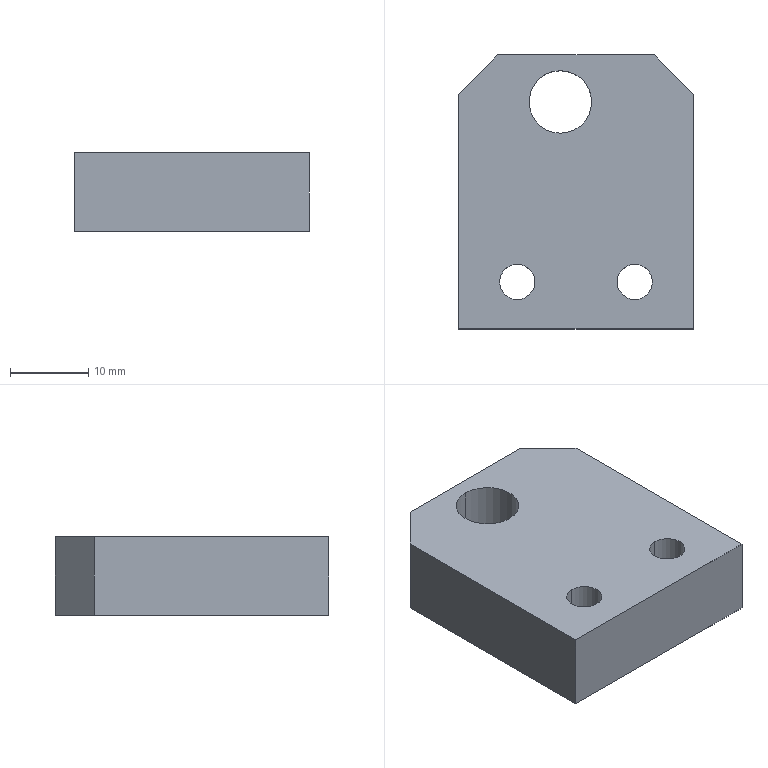Component | SolidWorks | LSDH-6-029-1 | 1 solid | 20 faces | box 30 x 35 x 10 mm | volume 9113 mm3 | cylinder 10 | plane 10 | commonest cylinder face diameters 8 x6 4.5 x4
build123d program:
from build123d import *

# Parameters (mm, degrees)
SKETCH1_W                                            = 35
SKETCH1_H                                            = 30
BOSS_EXTRUDE1_DEPTH                                  = 10
M8X1_0_TAPPED_HOLE1_D                                = 8
M8X1_0_TAPPED_HOLE1_DEPTH                            = 19
M8X1_0_TAPPED_HOLE1_TIP                              = 2.403
HOLE_SIZE_ACCORDING_TO_THE_TYPE_OF_HEX_S_D           = 4.5
HOLE_SIZE_ACCORDING_TO_THE_TYPE_OF_HEX_S_CBORE_D     = 8
HOLE_SIZE_ACCORDING_TO_THE_TYPE_OF_HEX_S_CBORE_DEPTH = 4.6
CHAMFER1_SIZE                                        = 5


with BuildPart() as part:
    # Sketch1 → Boss-Extrude1 (new body)
    with BuildSketch(Plane.XY):
        Rectangle(SKETCH1_W, SKETCH1_H)
    extrude(amount=BOSS_EXTRUDE1_DEPTH)

    # M8x1.0 Tapped Hole1
    with Locations(Plane(origin=(11.5, 2, 10), x_dir=(1, 0, 0), z_dir=(0, 0, 1))):
        with Locations((0, 0)):
            Hole(M8X1_0_TAPPED_HOLE1_D / 2, depth=M8X1_0_TAPPED_HOLE1_DEPTH)
            with Locations((0, 0, -(M8X1_0_TAPPED_HOLE1_DEPTH + M8X1_0_TAPPED_HOLE1_TIP / 2))):  # 118° drill point
                Cone(0, M8X1_0_TAPPED_HOLE1_D / 2, M8X1_0_TAPPED_HOLE1_TIP, mode=Mode.SUBTRACT)

    # Hole size according to the type of hex s (through all)
    with Locations(Plane(origin=(-11.5, 7.5, 0), x_dir=(-1, 0, 0), z_dir=(0, 0, -1))):
        with Locations((0, 0), (0, -15)):
            CounterBoreHole(HOLE_SIZE_ACCORDING_TO_THE_TYPE_OF_HEX_S_D / 2, HOLE_SIZE_ACCORDING_TO_THE_TYPE_OF_HEX_S_CBORE_D / 2, HOLE_SIZE_ACCORDING_TO_THE_TYPE_OF_HEX_S_CBORE_DEPTH)

    # Chamfer1
    chamfer1_edges = [part.edges().sort_by_distance(p)[0] for p in [
        (17.5, -15, 5),
        (17.5, 15, 5),
    ]]
    chamfer(chamfer1_edges, length=CHAMFER1_SIZE)


solid = part.part

# Placed as in the assembly
solid = solid.moved(Location((274.305, 297.675, 54.479), (0, 0, 90)))
STEP:
#1=COLOUR_RGB('',0.7922,0.8196,0.9333);
#2=FILL_AREA_STYLE_COLOUR('',#1);
#3=FILL_AREA_STYLE('',(#2));
#4=SURFACE_STYLE_FILL_AREA(#3);
#5=SURFACE_SIDE_STYLE('',(#4));
#6=SURFACE_STYLE_USAGE(.BOTH.,#5);
#7=PRESENTATION_STYLE_ASSIGNMENT((#6));
#8=CARTESIAN_POINT('',(10.504,11.424,2.326));
#9=VERTEX_POINT('',#8);
#10=CARTESIAN_POINT('',(10.504,11.109,2.326));
#11=VERTEX_POINT('',#10);
#12=CARTESIAN_POINT('',(10.504,11.267,2.326));
#13=DIRECTION('',(0.,-0.,-1.));
#14=DIRECTION('',(0.,-1.,0.));
#15=AXIS2_PLACEMENT_3D('',#12,#13,#14);
#16=CIRCLE('',#15,0.1575);
#17=EDGE_CURVE('',#9,#11,#16,.T.);
#18=ORIENTED_EDGE('',*,*,#17,.F.);
#19=CARTESIAN_POINT('',(10.504,11.424,2.145));
#20=VERTEX_POINT('',#19);
#21=CARTESIAN_POINT('',(10.504,11.424,2.145));
#22=DIRECTION('',(0.,-0.,-1.));
#23=VECTOR('',#22,39.37);
#24=LINE('',#21,#23);
#25=EDGE_CURVE('',#9,#20,#24,.T.);
#26=ORIENTED_EDGE('',*,*,#25,.T.);
#27=CARTESIAN_POINT('',(10.504,11.109,2.145));
#28=VERTEX_POINT('',#27);
#29=CARTESIAN_POINT('',(10.504,11.267,2.145));
#30=DIRECTION('',(0.,-0.,-1.));
#31=DIRECTION('',(0.,-1.,0.));
#32=AXIS2_PLACEMENT_3D('',#29,#30,#31);
#33=CIRCLE('',#32,0.1575);
#34=EDGE_CURVE('',#20,#28,#33,.T.);
#35=ORIENTED_EDGE('',*,*,#34,.T.);
#36=CARTESIAN_POINT('',(10.504,11.109,2.145));
#37=DIRECTION('',(0.,-0.,-1.));
#38=VECTOR('',#37,39.37);
#39=LINE('',#36,#38);
#40=EDGE_CURVE('',#11,#28,#39,.T.);
#41=ORIENTED_EDGE('',*,*,#40,.F.);
#42=EDGE_LOOP('',(#18,#26,#35,#41));
#43=FACE_OUTER_BOUND('',#42,.T.);
#44=CARTESIAN_POINT('',(10.504,11.267,2.145));
#45=DIRECTION('',(0.,-0.,-1.));
#46=DIRECTION('',(0.,-1.,0.));
#47=AXIS2_PLACEMENT_3D('',#44,#45,#46);
#48=CYLINDRICAL_SURFACE('',#47,0.1575);
#49=ADVANCED_FACE('',(#43),#48,.F.);
#50=CARTESIAN_POINT('',(10.504,11.355,2.539));
#51=VERTEX_POINT('',#50);
#52=CARTESIAN_POINT('',(10.504,11.178,2.539));
#53=VERTEX_POINT('',#52);
#54=CARTESIAN_POINT('',(10.504,11.267,2.539));
#55=DIRECTION('',(0.,-0.,-1.));
#56=DIRECTION('',(0.,-1.,0.));
#57=AXIS2_PLACEMENT_3D('',#54,#55,#56);
#58=CIRCLE('',#57,0.08858);
#59=EDGE_CURVE('',#51,#53,#58,.T.);
#60=ORIENTED_EDGE('',*,*,#59,.F.);
#61=CARTESIAN_POINT('',(10.504,11.355,2.326));
#62=VERTEX_POINT('',#61);
#63=CARTESIAN_POINT('',(10.504,11.355,2.145));
#64=DIRECTION('',(0.,-0.,-1.));
#65=VECTOR('',#64,39.37);
#66=LINE('',#63,#65);
#67=EDGE_CURVE('',#51,#62,#66,.T.);
#68=ORIENTED_EDGE('',*,*,#67,.T.);
#69=CARTESIAN_POINT('',(10.504,11.178,2.326));
#70=VERTEX_POINT('',#69);
#71=CARTESIAN_POINT('',(10.504,11.267,2.326));
#72=DIRECTION('',(0.,-0.,-1.));
#73=DIRECTION('',(0.,-1.,0.));
#74=AXIS2_PLACEMENT_3D('',#71,#72,#73);
#75=CIRCLE('',#74,0.08858);
#76=EDGE_CURVE('',#62,#70,#75,.T.);
#77=ORIENTED_EDGE('',*,*,#76,.T.);
#78=CARTESIAN_POINT('',(10.504,11.178,2.145));
#79=DIRECTION('',(0.,-0.,-1.));
#80=VECTOR('',#79,39.37);
#81=LINE('',#78,#80);
#82=EDGE_CURVE('',#53,#70,#81,.T.);
#83=ORIENTED_EDGE('',*,*,#82,.F.);
#84=EDGE_LOOP('',(#60,#68,#77,#83));
#85=FACE_OUTER_BOUND('',#84,.T.);
#86=CARTESIAN_POINT('',(10.504,11.267,2.145));
#87=DIRECTION('',(0.,-0.,-1.));
#88=DIRECTION('',(0.,-1.,0.));
#89=AXIS2_PLACEMENT_3D('',#86,#87,#88);
#90=CYLINDRICAL_SURFACE('',#89,0.08858);
#91=ADVANCED_FACE('',(#85),#90,.F.);
#92=CARTESIAN_POINT('',(11.095,11.424,2.326));
#93=VERTEX_POINT('',#92);
#94=CARTESIAN_POINT('',(11.095,11.109,2.326));
#95=VERTEX_POINT('',#94);
#96=CARTESIAN_POINT('',(11.095,11.267,2.326));
#97=DIRECTION('',(0.,-0.,-1.));
#98=DIRECTION('',(0.,-1.,0.));
#99=AXIS2_PLACEMENT_3D('',#96,#97,#98);
#100=CIRCLE('',#99,0.1575);
#101=EDGE_CURVE('',#93,#95,#100,.T.);
#102=ORIENTED_EDGE('',*,*,#101,.F.);
#103=CARTESIAN_POINT('',(11.095,11.424,2.145));
#104=VERTEX_POINT('',#103);
#105=CARTESIAN_POINT('',(11.095,11.424,2.145));
#106=DIRECTION('',(0.,-0.,-1.));
#107=VECTOR('',#106,39.37);
#108=LINE('',#105,#107);
#109=EDGE_CURVE('',#93,#104,#108,.T.);
#110=ORIENTED_EDGE('',*,*,#109,.T.);
#111=CARTESIAN_POINT('',(11.095,11.109,2.145));
#112=VERTEX_POINT('',#111);
#113=CARTESIAN_POINT('',(11.095,11.267,2.145));
#114=DIRECTION('',(0.,-0.,-1.));
#115=DIRECTION('',(0.,-1.,0.));
#116=AXIS2_PLACEMENT_3D('',#113,#114,#115);
#117=CIRCLE('',#116,0.1575);
#118=EDGE_CURVE('',#104,#112,#117,.T.);
#119=ORIENTED_EDGE('',*,*,#118,.T.);
#120=CARTESIAN_POINT('',(11.095,11.109,2.145));
#121=DIRECTION('',(0.,-0.,-1.));
#122=VECTOR('',#121,39.37);
#123=LINE('',#120,#122);
#124=EDGE_CURVE('',#95,#112,#123,.T.);
#125=ORIENTED_EDGE('',*,*,#124,.F.);
#126=EDGE_LOOP('',(#102,#110,#119,#125));
#127=FACE_OUTER_BOUND('',#126,.T.);
#128=CARTESIAN_POINT('',(11.095,11.267,2.145));
#129=DIRECTION('',(0.,-0.,-1.));
#130=DIRECTION('',(0.,-1.,0.));
#131=AXIS2_PLACEMENT_3D('',#128,#129,#130);
#132=CYLINDRICAL_SURFACE('',#131,0.1575);
#133=ADVANCED_FACE('',(#127),#132,.F.);
#134=CARTESIAN_POINT('',(11.095,11.355,2.539));
#135=VERTEX_POINT('',#134);
#136=CARTESIAN_POINT('',(11.095,11.178,2.539));
#137=VERTEX_POINT('',#136);
#138=CARTESIAN_POINT('',(11.095,11.267,2.539));
#139=DIRECTION('',(0.,-0.,-1.));
#140=DIRECTION('',(0.,-1.,0.));
#141=AXIS2_PLACEMENT_3D('',#138,#139,#140);
#142=CIRCLE('',#141,0.08858);
#143=EDGE_CURVE('',#135,#137,#142,.T.);
#144=ORIENTED_EDGE('',*,*,#143,.F.);
#145=CARTESIAN_POINT('',(11.095,11.355,2.326));
#146=VERTEX_POINT('',#145);
#147=CARTESIAN_POINT('',(11.095,11.355,2.145));
#148=DIRECTION('',(0.,-0.,-1.));
#149=VECTOR('',#148,39.37);
#150=LINE('',#147,#149);
#151=EDGE_CURVE('',#135,#146,#150,.T.);
#152=ORIENTED_EDGE('',*,*,#151,.T.);
#153=CARTESIAN_POINT('',(11.095,11.178,2.326));
#154=VERTEX_POINT('',#153);
#155=CARTESIAN_POINT('',(11.095,11.267,2.326));
#156=DIRECTION('',(0.,-0.,-1.));
#157=DIRECTION('',(0.,-1.,0.));
#158=AXIS2_PLACEMENT_3D('',#155,#156,#157);
#159=CIRCLE('',#158,0.08858);
#160=EDGE_CURVE('',#146,#154,#159,.T.);
#161=ORIENTED_EDGE('',*,*,#160,.T.);
#162=CARTESIAN_POINT('',(11.095,11.178,2.145));
#163=DIRECTION('',(0.,-0.,-1.));
#164=VECTOR('',#163,39.37);
#165=LINE('',#162,#164);
#166=EDGE_CURVE('',#137,#154,#165,.T.);
#167=ORIENTED_EDGE('',*,*,#166,.F.);
#168=EDGE_LOOP('',(#144,#152,#161,#167));
#169=FACE_OUTER_BOUND('',#168,.T.);
#170=CARTESIAN_POINT('',(11.095,11.267,2.145));
#171=DIRECTION('',(0.,-0.,-1.));
#172=DIRECTION('',(0.,-1.,0.));
#173=AXIS2_PLACEMENT_3D('',#170,#171,#172);
#174=CYLINDRICAL_SURFACE('',#173,0.08858);
#175=ADVANCED_FACE('',(#169),#174,.F.);
#176=CARTESIAN_POINT('',(10.721,12.015,2.145));
#177=VERTEX_POINT('',#176);
#178=CARTESIAN_POINT('',(10.721,12.33,2.145));
#179=VERTEX_POINT('',#178);
#180=CARTESIAN_POINT('',(10.721,12.172,2.145));
#181=DIRECTION('',(-0.,0.,1.));
#182=DIRECTION('',(0.,1.,0.));
#183=AXIS2_PLACEMENT_3D('',#180,#181,#182);
#184=CIRCLE('',#183,0.1575);
#185=EDGE_CURVE('',#177,#179,#184,.T.);
#186=ORIENTED_EDGE('',*,*,#185,.F.);
#187=CARTESIAN_POINT('',(10.721,12.015,2.539));
#188=VERTEX_POINT('',#187);
#189=CARTESIAN_POINT('',(10.721,12.015,2.539));
#190=DIRECTION('',(-0.,0.,1.));
#191=VECTOR('',#190,39.37);
#192=LINE('',#189,#191);
#193=EDGE_CURVE('',#177,#188,#192,.T.);
#194=ORIENTED_EDGE('',*,*,#193,.T.);
#195=CARTESIAN_POINT('',(10.721,12.33,2.539));
#196=VERTEX_POINT('',#195);
#197=CARTESIAN_POINT('',(10.721,12.172,2.539));
#198=DIRECTION('',(-0.,0.,1.));
#199=DIRECTION('',(0.,1.,0.));
#200=AXIS2_PLACEMENT_3D('',#197,#198,#199);
#201=CIRCLE('',#200,0.1575);
#202=EDGE_CURVE('',#188,#196,#201,.T.);
#203=ORIENTED_EDGE('',*,*,#202,.T.);
#204=CARTESIAN_POINT('',(10.721,12.33,2.539));
#205=DIRECTION('',(-0.,0.,1.));
#206=VECTOR('',#205,39.37);
#207=LINE('',#204,#206);
#208=EDGE_CURVE('',#179,#196,#207,.T.);
#209=ORIENTED_EDGE('',*,*,#208,.F.);
#210=EDGE_LOOP('',(#186,#194,#203,#209));
#211=FACE_OUTER_BOUND('',#210,.T.);
#212=CARTESIAN_POINT('',(10.721,12.172,2.539));
#213=DIRECTION('',(-0.,0.,1.));
#214=DIRECTION('',(0.,1.,0.));
#215=AXIS2_PLACEMENT_3D('',#212,#213,#214);
#216=CYLINDRICAL_SURFACE('',#215,0.1575);
#217=ADVANCED_FACE('',(#211),#216,.F.);
#218=CARTESIAN_POINT('',(11.193,12.408,2.539));
#219=VERTEX_POINT('',#218);
#220=CARTESIAN_POINT('',(10.406,12.408,2.539));
#221=VERTEX_POINT('',#220);
#222=CARTESIAN_POINT('',(10.209,12.408,2.539));
#223=DIRECTION('',(-1.,-0.,-0.));
#224=VECTOR('',#223,39.37);
#225=LINE('',#222,#224);
#226=EDGE_CURVE('',#219,#221,#225,.T.);
#227=ORIENTED_EDGE('',*,*,#226,.F.);
#228=CARTESIAN_POINT('',(11.193,12.408,2.145));
#229=VERTEX_POINT('',#228);
#230=CARTESIAN_POINT('',(11.193,12.408,2.539));
#231=DIRECTION('',(0.,-0.,-1.));
#232=VECTOR('',#231,39.37);
#233=LINE('',#230,#232);
#234=EDGE_CURVE('',#219,#229,#233,.T.);
#235=ORIENTED_EDGE('',*,*,#234,.T.);
#236=CARTESIAN_POINT('',(10.406,12.408,2.145));
#237=VERTEX_POINT('',#236);
#238=CARTESIAN_POINT('',(10.209,12.408,2.145));
#239=DIRECTION('',(-1.,-0.,-0.));
#240=VECTOR('',#239,39.37);
#241=LINE('',#238,#240);
#242=EDGE_CURVE('',#229,#237,#241,.T.);
#243=ORIENTED_EDGE('',*,*,#242,.T.);
#244=CARTESIAN_POINT('',(10.406,12.408,2.539));
#245=DIRECTION('',(-0.,0.,1.));
#246=VECTOR('',#245,39.37);
#247=LINE('',#244,#246);
#248=EDGE_CURVE('',#237,#221,#247,.T.);
#249=ORIENTED_EDGE('',*,*,#248,.T.);
#250=EDGE_LOOP('',(#227,#235,#243,#249));
#251=FACE_OUTER_BOUND('',#250,.T.);
#252=CARTESIAN_POINT('',(10.209,12.408,2.539));
#253=DIRECTION('',(0.,-1.,0.));
#254=DIRECTION('',(1.,0.,0.));
#255=AXIS2_PLACEMENT_3D('',#252,#253,#254);
#256=PLANE('',#255);
#257=ADVANCED_FACE('',(#251),#256,.F.);
#258=CARTESIAN_POINT('',(10.209,12.212,2.539));
#259=VERTEX_POINT('',#258);
#260=CARTESIAN_POINT('',(10.209,11.031,2.539));
#261=VERTEX_POINT('',#260);
#262=CARTESIAN_POINT('',(10.209,11.031,2.539));
#263=DIRECTION('',(-0.,-1.,0.));
#264=VECTOR('',#263,39.37);
#265=LINE('',#262,#264);
#266=EDGE_CURVE('',#259,#261,#265,.T.);
#267=ORIENTED_EDGE('',*,*,#266,.F.);
#268=CARTESIAN_POINT('',(10.209,12.212,2.145));
#269=VERTEX_POINT('',#268);
#270=CARTESIAN_POINT('',(10.209,12.212,2.539));
#271=DIRECTION('',(0.,-0.,-1.));
#272=VECTOR('',#271,39.37);
#273=LINE('',#270,#272);
#274=EDGE_CURVE('',#259,#269,#273,.T.);
#275=ORIENTED_EDGE('',*,*,#274,.T.);
#276=CARTESIAN_POINT('',(10.209,11.031,2.145));
#277=VERTEX_POINT('',#276);
#278=CARTESIAN_POINT('',(10.209,11.031,2.145));
#279=DIRECTION('',(-0.,-1.,0.));
#280=VECTOR('',#279,39.37);
#281=LINE('',#278,#280);
#282=EDGE_CURVE('',#269,#277,#281,.T.);
#283=ORIENTED_EDGE('',*,*,#282,.T.);
#284=CARTESIAN_POINT('',(10.209,11.031,2.539));
#285=DIRECTION('',(0.,-0.,-1.));
#286=VECTOR('',#285,39.37);
#287=LINE('',#284,#286);
#288=EDGE_CURVE('',#261,#277,#287,.T.);
#289=ORIENTED_EDGE('',*,*,#288,.F.);
#290=EDGE_LOOP('',(#267,#275,#283,#289));
#291=FACE_OUTER_BOUND('',#290,.T.);
#292=CARTESIAN_POINT('',(10.209,11.031,2.539));
#293=DIRECTION('',(1.,-0.,0.));
#294=DIRECTION('',(0.,-0.,-1.));
#295=AXIS2_PLACEMENT_3D('',#292,#293,#294);
#296=PLANE('',#295);
#297=ADVANCED_FACE('',(#291),#296,.F.);
#298=CARTESIAN_POINT('',(11.39,11.031,2.145));
#299=VERTEX_POINT('',#298);
#300=CARTESIAN_POINT('',(10.209,11.031,2.145));
#301=DIRECTION('',(1.,0.,0.));
#302=VECTOR('',#301,39.37);
#303=LINE('',#300,#302);
#304=EDGE_CURVE('',#277,#299,#303,.T.);
#305=ORIENTED_EDGE('',*,*,#304,.T.);
#306=CARTESIAN_POINT('',(11.39,11.031,2.539));
#307=VERTEX_POINT('',#306);
#308=CARTESIAN_POINT('',(11.39,11.031,2.539));
#309=DIRECTION('',(0.,-0.,-1.));
#310=VECTOR('',#309,39.37);
#311=LINE('',#308,#310);
#312=EDGE_CURVE('',#307,#299,#311,.T.);
#313=ORIENTED_EDGE('',*,*,#312,.F.);
#314=CARTESIAN_POINT('',(10.209,11.031,2.539));
#315=DIRECTION('',(1.,0.,0.));
#316=VECTOR('',#315,39.37);
#317=LINE('',#314,#316);
#318=EDGE_CURVE('',#261,#307,#317,.T.);
#319=ORIENTED_EDGE('',*,*,#318,.F.);
#320=ORIENTED_EDGE('',*,*,#288,.T.);
#321=EDGE_LOOP('',(#305,#313,#319,#320));
#322=FACE_OUTER_BOUND('',#321,.T.);
#323=CARTESIAN_POINT('',(10.209,11.031,2.539));
#324=DIRECTION('',(-0.,1.,-0.));
#325=DIRECTION('',(-1.,-0.,-0.));
#326=AXIS2_PLACEMENT_3D('',#323,#324,#325);
#327=PLANE('',#326);
#328=ADVANCED_FACE('',(#322),#327,.F.);
#329=CARTESIAN_POINT('',(11.39,12.212,2.145));
#330=VERTEX_POINT('',#329);
#331=CARTESIAN_POINT('',(11.39,11.031,2.145));
#332=DIRECTION('',(0.,1.,-0.));
#333=VECTOR('',#332,39.37);
#334=LINE('',#331,#333);
#335=EDGE_CURVE('',#299,#330,#334,.T.);
#336=ORIENTED_EDGE('',*,*,#335,.T.);
#337=CARTESIAN_POINT('',(11.39,12.212,2.539));
#338=VERTEX_POINT('',#337);
#339=CARTESIAN_POINT('',(11.39,12.212,2.539));
#340=DIRECTION('',(-0.,0.,1.));
#341=VECTOR('',#340,39.37);
#342=LINE('',#339,#341);
#343=EDGE_CURVE('',#330,#338,#342,.T.);
#344=ORIENTED_EDGE('',*,*,#343,.T.);
#345=CARTESIAN_POINT('',(11.39,11.031,2.539));
#346=DIRECTION('',(0.,1.,-0.));
#347=VECTOR('',#346,39.37);
#348=LINE('',#345,#347);
#349=EDGE_CURVE('',#307,#338,#348,.T.);
#350=ORIENTED_EDGE('',*,*,#349,.F.);
#351=ORIENTED_EDGE('',*,*,#312,.T.);
#352=EDGE_LOOP('',(#336,#344,#350,#351));
#353=FACE_OUTER_BOUND('',#352,.T.);
#354=CARTESIAN_POINT('',(11.39,11.031,2.539));
#355=DIRECTION('',(-1.,0.,-0.));
#356=DIRECTION('',(-0.,0.,1.));
#357=AXIS2_PLACEMENT_3D('',#354,#355,#356);
#358=PLANE('',#357);
#359=ADVANCED_FACE('',(#353),#358,.F.);
#360=CARTESIAN_POINT('',(10.504,11.267,2.539));
#361=DIRECTION('',(0.,-0.,-1.));
#362=DIRECTION('',(0.,-1.,0.));
#363=AXIS2_PLACEMENT_3D('',#360,#361,#362);
#364=CIRCLE('',#363,0.08858);
#365=EDGE_CURVE('',#53,#51,#364,.T.);
#366=ORIENTED_EDGE('',*,*,#365,.T.);
#367=ORIENTED_EDGE('',*,*,#59,.T.);
#368=EDGE_LOOP('',(#366,#367));
#369=FACE_BOUND('',#368,.T.);
#370=CARTESIAN_POINT('',(11.095,11.267,2.539));
#371=DIRECTION('',(0.,-0.,-1.));
#372=DIRECTION('',(0.,-1.,0.));
#373=AXIS2_PLACEMENT_3D('',#370,#371,#372);
#374=CIRCLE('',#373,0.08858);
#375=EDGE_CURVE('',#137,#135,#374,.T.);
#376=ORIENTED_EDGE('',*,*,#375,.T.);
#377=ORIENTED_EDGE('',*,*,#143,.T.);
#378=EDGE_LOOP('',(#376,#377));
#379=FACE_BOUND('',#378,.T.);
#380=CARTESIAN_POINT('',(10.721,12.172,2.539));
#381=DIRECTION('',(-0.,0.,1.));
#382=DIRECTION('',(0.,1.,0.));
#383=AXIS2_PLACEMENT_3D('',#380,#381,#382);
#384=CIRCLE('',#383,0.1575);
#385=EDGE_CURVE('',#196,#188,#384,.T.);
#386=ORIENTED_EDGE('',*,*,#385,.F.);
#387=ORIENTED_EDGE('',*,*,#202,.F.);
#388=EDGE_LOOP('',(#386,#387));
#389=FACE_BOUND('',#388,.T.);
#390=ORIENTED_EDGE('',*,*,#349,.T.);
#391=CARTESIAN_POINT('',(11.341,12.261,2.539));
#392=DIRECTION('',(-0.7071,0.7071,-0.));
#393=VECTOR('',#392,39.37);
#394=LINE('',#391,#393);
#395=EDGE_CURVE('',#338,#219,#394,.T.);
#396=ORIENTED_EDGE('',*,*,#395,.T.);
#397=ORIENTED_EDGE('',*,*,#226,.T.);
#398=CARTESIAN_POINT('',(10.258,12.261,2.539));
#399=DIRECTION('',(-0.7071,-0.7071,-0.));
#400=VECTOR('',#399,39.37);
#401=LINE('',#398,#400);
#402=EDGE_CURVE('',#221,#259,#401,.T.);
#403=ORIENTED_EDGE('',*,*,#402,.T.);
#404=ORIENTED_EDGE('',*,*,#266,.T.);
#405=ORIENTED_EDGE('',*,*,#318,.T.);
#406=EDGE_LOOP('',(#390,#396,#397,#403,#404,#405));
#407=FACE_OUTER_BOUND('',#406,.T.);
#408=CARTESIAN_POINT('',(10.799,11.72,2.539));
#409=DIRECTION('',(-0.,0.,1.));
#410=DIRECTION('',(0.,1.,-0.));
#411=AXIS2_PLACEMENT_3D('',#408,#409,#410);
#412=PLANE('',#411);
#413=ADVANCED_FACE('',(#369,#379,#389,#407),#412,.T.);
#414=CARTESIAN_POINT('',(10.504,11.267,2.145));
#415=DIRECTION('',(0.,-0.,-1.));
#416=DIRECTION('',(0.,-1.,0.));
#417=AXIS2_PLACEMENT_3D('',#414,#415,#416);
#418=CIRCLE('',#417,0.1575);
#419=EDGE_CURVE('',#28,#20,#418,.T.);
#420=ORIENTED_EDGE('',*,*,#419,.F.);
#421=ORIENTED_EDGE('',*,*,#34,.F.);
#422=EDGE_LOOP('',(#420,#421));
#423=FACE_BOUND('',#422,.T.);
#424=CARTESIAN_POINT('',(11.095,11.267,2.145));
#425=DIRECTION('',(0.,-0.,-1.));
#426=DIRECTION('',(0.,-1.,0.));
#427=AXIS2_PLACEMENT_3D('',#424,#425,#426);
#428=CIRCLE('',#427,0.1575);
#429=EDGE_CURVE('',#112,#104,#428,.T.);
#430=ORIENTED_EDGE('',*,*,#429,.F.);
#431=ORIENTED_EDGE('',*,*,#118,.F.);
#432=EDGE_LOOP('',(#430,#431));
#433=FACE_BOUND('',#432,.T.);
#434=CARTESIAN_POINT('',(10.721,12.172,2.145));
#435=DIRECTION('',(-0.,0.,1.));
#436=DIRECTION('',(0.,1.,0.));
#437=AXIS2_PLACEMENT_3D('',#434,#435,#436);
#438=CIRCLE('',#437,0.1575);
#439=EDGE_CURVE('',#179,#177,#438,.T.);
#440=ORIENTED_EDGE('',*,*,#439,.T.);
#441=ORIENTED_EDGE('',*,*,#185,.T.);
#442=EDGE_LOOP('',(#440,#441));
#443=FACE_BOUND('',#442,.T.);
#444=ORIENTED_EDGE('',*,*,#242,.F.);
#445=CARTESIAN_POINT('',(11.193,12.408,2.145));
#446=DIRECTION('',(0.7071,-0.7071,0.));
#447=VECTOR('',#446,39.37);
#448=LINE('',#445,#447);
#449=EDGE_CURVE('',#229,#330,#448,.T.);
#450=ORIENTED_EDGE('',*,*,#449,.T.);
#451=ORIENTED_EDGE('',*,*,#335,.F.);
#452=ORIENTED_EDGE('',*,*,#304,.F.);
#453=ORIENTED_EDGE('',*,*,#282,.F.);
#454=CARTESIAN_POINT('',(10.209,12.212,2.145));
#455=DIRECTION('',(0.7071,0.7071,0.));
#456=VECTOR('',#455,39.37);
#457=LINE('',#454,#456);
#458=EDGE_CURVE('',#269,#237,#457,.T.);
#459=ORIENTED_EDGE('',*,*,#458,.T.);
#460=EDGE_LOOP('',(#444,#450,#451,#452,#453,#459));
#461=FACE_OUTER_BOUND('',#460,.T.);
#462=CARTESIAN_POINT('',(10.799,11.72,2.145));
#463=DIRECTION('',(-0.,0.,1.));
#464=DIRECTION('',(0.,1.,-0.));
#465=AXIS2_PLACEMENT_3D('',#462,#463,#464);
#466=PLANE('',#465);
#467=ADVANCED_FACE('',(#423,#433,#443,#461),#466,.F.);
#468=ORIENTED_EDGE('',*,*,#193,.F.);
#469=ORIENTED_EDGE('',*,*,#439,.F.);
#470=ORIENTED_EDGE('',*,*,#208,.T.);
#471=ORIENTED_EDGE('',*,*,#385,.T.);
#472=EDGE_LOOP('',(#468,#469,#470,#471));
#473=FACE_OUTER_BOUND('',#472,.T.);
#474=CARTESIAN_POINT('',(10.721,12.172,2.539));
#475=DIRECTION('',(-0.,0.,1.));
#476=DIRECTION('',(0.,1.,0.));
#477=AXIS2_PLACEMENT_3D('',#474,#475,#476);
#478=CYLINDRICAL_SURFACE('',#477,0.1575);
#479=ADVANCED_FACE('',(#473),#478,.F.);
#480=ORIENTED_EDGE('',*,*,#151,.F.);
#481=ORIENTED_EDGE('',*,*,#375,.F.);
#482=ORIENTED_EDGE('',*,*,#166,.T.);
#483=CARTESIAN_POINT('',(11.095,11.267,2.326));
#484=DIRECTION('',(0.,-0.,-1.));
#485=DIRECTION('',(0.,-1.,0.));
#486=AXIS2_PLACEMENT_3D('',#483,#484,#485);
#487=CIRCLE('',#486,0.08858);
#488=EDGE_CURVE('',#154,#146,#487,.T.);
#489=ORIENTED_EDGE('',*,*,#488,.T.);
#490=EDGE_LOOP('',(#480,#481,#482,#489));
#491=FACE_OUTER_BOUND('',#490,.T.);
#492=CARTESIAN_POINT('',(11.095,11.267,2.145));
#493=DIRECTION('',(0.,-0.,-1.));
#494=DIRECTION('',(0.,-1.,0.));
#495=AXIS2_PLACEMENT_3D('',#492,#493,#494);
#496=CYLINDRICAL_SURFACE('',#495,0.08858);
#497=ADVANCED_FACE('',(#491),#496,.F.);
#498=ORIENTED_EDGE('',*,*,#488,.F.);
#499=ORIENTED_EDGE('',*,*,#160,.F.);
#500=EDGE_LOOP('',(#498,#499));
#501=FACE_BOUND('',#500,.T.);
#502=CARTESIAN_POINT('',(11.095,11.267,2.326));
#503=DIRECTION('',(0.,-0.,-1.));
#504=DIRECTION('',(0.,-1.,0.));
#505=AXIS2_PLACEMENT_3D('',#502,#503,#504);
#506=CIRCLE('',#505,0.1575);
#507=EDGE_CURVE('',#95,#93,#506,.T.);
#508=ORIENTED_EDGE('',*,*,#507,.T.);
#509=ORIENTED_EDGE('',*,*,#101,.T.);
#510=EDGE_LOOP('',(#508,#509));
#511=FACE_OUTER_BOUND('',#510,.T.);
#512=CARTESIAN_POINT('',(11.095,11.355,2.326));
#513=DIRECTION('',(-0.,0.,1.));
#514=DIRECTION('',(0.,1.,-0.));
#515=AXIS2_PLACEMENT_3D('',#512,#513,#514);
#516=PLANE('',#515);
#517=ADVANCED_FACE('',(#501,#511),#516,.F.);
#518=ORIENTED_EDGE('',*,*,#109,.F.);
#519=ORIENTED_EDGE('',*,*,#507,.F.);
#520=ORIENTED_EDGE('',*,*,#124,.T.);
#521=ORIENTED_EDGE('',*,*,#429,.T.);
#522=EDGE_LOOP('',(#518,#519,#520,#521));
#523=FACE_OUTER_BOUND('',#522,.T.);
#524=CARTESIAN_POINT('',(11.095,11.267,2.145));
#525=DIRECTION('',(0.,-0.,-1.));
#526=DIRECTION('',(0.,-1.,0.));
#527=AXIS2_PLACEMENT_3D('',#524,#525,#526);
#528=CYLINDRICAL_SURFACE('',#527,0.1575);
#529=ADVANCED_FACE('',(#523),#528,.F.);
#530=ORIENTED_EDGE('',*,*,#67,.F.);
#531=ORIENTED_EDGE('',*,*,#365,.F.);
#532=ORIENTED_EDGE('',*,*,#82,.T.);
#533=CARTESIAN_POINT('',(10.504,11.267,2.326));
#534=DIRECTION('',(0.,-0.,-1.));
#535=DIRECTION('',(0.,-1.,0.));
#536=AXIS2_PLACEMENT_3D('',#533,#534,#535);
#537=CIRCLE('',#536,0.08858);
#538=EDGE_CURVE('',#70,#62,#537,.T.);
#539=ORIENTED_EDGE('',*,*,#538,.T.);
#540=EDGE_LOOP('',(#530,#531,#532,#539));
#541=FACE_OUTER_BOUND('',#540,.T.);
#542=CARTESIAN_POINT('',(10.504,11.267,2.145));
#543=DIRECTION('',(0.,-0.,-1.));
#544=DIRECTION('',(0.,-1.,0.));
#545=AXIS2_PLACEMENT_3D('',#542,#543,#544);
#546=CYLINDRICAL_SURFACE('',#545,0.08858);
#547=ADVANCED_FACE('',(#541),#546,.F.);
#548=ORIENTED_EDGE('',*,*,#538,.F.);
#549=ORIENTED_EDGE('',*,*,#76,.F.);
#550=EDGE_LOOP('',(#548,#549));
#551=FACE_BOUND('',#550,.T.);
#552=CARTESIAN_POINT('',(10.504,11.267,2.326));
#553=DIRECTION('',(0.,-0.,-1.));
#554=DIRECTION('',(0.,-1.,0.));
#555=AXIS2_PLACEMENT_3D('',#552,#553,#554);
#556=CIRCLE('',#555,0.1575);
#557=EDGE_CURVE('',#11,#9,#556,.T.);
#558=ORIENTED_EDGE('',*,*,#557,.T.);
#559=ORIENTED_EDGE('',*,*,#17,.T.);
#560=EDGE_LOOP('',(#558,#559));
#561=FACE_OUTER_BOUND('',#560,.T.);
#562=CARTESIAN_POINT('',(10.504,11.355,2.326));
#563=DIRECTION('',(-0.,0.,1.));
#564=DIRECTION('',(0.,1.,-0.));
#565=AXIS2_PLACEMENT_3D('',#562,#563,#564);
#566=PLANE('',#565);
#567=ADVANCED_FACE('',(#551,#561),#566,.F.);
#568=ORIENTED_EDGE('',*,*,#25,.F.);
#569=ORIENTED_EDGE('',*,*,#557,.F.);
#570=ORIENTED_EDGE('',*,*,#40,.T.);
#571=ORIENTED_EDGE('',*,*,#419,.T.);
#572=EDGE_LOOP('',(#568,#569,#570,#571));
#573=FACE_OUTER_BOUND('',#572,.T.);
#574=CARTESIAN_POINT('',(10.504,11.267,2.145));
#575=DIRECTION('',(0.,-0.,-1.));
#576=DIRECTION('',(0.,-1.,0.));
#577=AXIS2_PLACEMENT_3D('',#574,#575,#576);
#578=CYLINDRICAL_SURFACE('',#577,0.1575);
#579=ADVANCED_FACE('',(#573),#578,.F.);
#580=ORIENTED_EDGE('',*,*,#395,.F.);
#581=ORIENTED_EDGE('',*,*,#343,.F.);
#582=ORIENTED_EDGE('',*,*,#449,.F.);
#583=ORIENTED_EDGE('',*,*,#234,.F.);
#584=EDGE_LOOP('',(#580,#581,#582,#583));
#585=FACE_OUTER_BOUND('',#584,.T.);
#586=CARTESIAN_POINT('',(11.193,12.408,2.539));
#587=DIRECTION('',(-0.7071,-0.7071,-0.));
#588=DIRECTION('',(0.,-0.,-1.));
#589=AXIS2_PLACEMENT_3D('',#586,#587,#588);
#590=PLANE('',#589);
#591=ADVANCED_FACE('',(#585),#590,.F.);
#592=ORIENTED_EDGE('',*,*,#402,.F.);
#593=ORIENTED_EDGE('',*,*,#248,.F.);
#594=ORIENTED_EDGE('',*,*,#458,.F.);
#595=ORIENTED_EDGE('',*,*,#274,.F.);
#596=EDGE_LOOP('',(#592,#593,#594,#595));
#597=FACE_OUTER_BOUND('',#596,.T.);
#598=CARTESIAN_POINT('',(10.209,12.212,2.539));
#599=DIRECTION('',(0.7071,-0.7071,0.));
#600=DIRECTION('',(0.,-0.,-1.));
#601=AXIS2_PLACEMENT_3D('',#598,#599,#600);
#602=PLANE('',#601);
#603=ADVANCED_FACE('',(#597),#602,.F.);
#604=CLOSED_SHELL('',(#49,#91,#133,#175,#217,#257,#297,#328,#359,#413,#467,#479,#497,#517,#529,#547,#567,#579,#591,#603));
#605=MANIFOLD_SOLID_BREP('',#604);
#606=STYLED_ITEM('',(#7),#605);
#607=PRESENTATION_LAYER_ASSIGNMENT('','',(#606));
#608=(LENGTH_UNIT()NAMED_UNIT(*)SI_UNIT($,.METRE.));
#609=LENGTH_MEASURE_WITH_UNIT(LENGTH_MEASURE(0.0254),#608);
#610=DIMENSIONAL_EXPONENTS(1.,0.,0.,0.,0.,0.,0.);
#611=(CONVERSION_BASED_UNIT('',#609)LENGTH_UNIT()NAMED_UNIT(#610));
#612=UNCERTAINTY_MEASURE_WITH_UNIT(LENGTH_MEASURE(0.00001),#611,'','');
#613=(NAMED_UNIT(*)PLANE_ANGLE_UNIT()SI_UNIT($,.RADIAN.));
#614=(NAMED_UNIT(*)SI_UNIT($,.STERADIAN.)SOLID_ANGLE_UNIT());
#615=(GEOMETRIC_REPRESENTATION_CONTEXT(3)GLOBAL_UNCERTAINTY_ASSIGNED_CONTEXT((#612))GLOBAL_UNIT_ASSIGNED_CONTEXT((#611,#613,#614))REPRESENTATION_CONTEXT('',''));
#616=MECHANICAL_DESIGN_GEOMETRIC_PRESENTATION_REPRESENTATION('',(#606),#615);
#617=CARTESIAN_POINT('',(0.,0.,0.));
#618=DIRECTION('',(0.,0.,1.));
#619=DIRECTION('',(1.,0.,0.));
#620=AXIS2_PLACEMENT_3D('',#617,#618,#619);
#621=(LENGTH_UNIT()NAMED_UNIT(*)SI_UNIT($,.METRE.));
#622=LENGTH_MEASURE_WITH_UNIT(LENGTH_MEASURE(0.0254),#621);
#623=DIMENSIONAL_EXPONENTS(1.,0.,0.,0.,0.,0.,0.);
#624=(CONVERSION_BASED_UNIT('',#622)LENGTH_UNIT()NAMED_UNIT(#623));
#625=UNCERTAINTY_MEASURE_WITH_UNIT(LENGTH_MEASURE(0.00001),#624,'','');
#626=(NAMED_UNIT(*)PLANE_ANGLE_UNIT()SI_UNIT($,.RADIAN.));
#627=(NAMED_UNIT(*)SI_UNIT($,.STERADIAN.)SOLID_ANGLE_UNIT());
#628=(GEOMETRIC_REPRESENTATION_CONTEXT(3)GLOBAL_UNCERTAINTY_ASSIGNED_CONTEXT((#625))GLOBAL_UNIT_ASSIGNED_CONTEXT((#624,#626,#627))REPRESENTATION_CONTEXT('',''));
#629=ADVANCED_BREP_SHAPE_REPRESENTATION('',(#605,#620),#628);